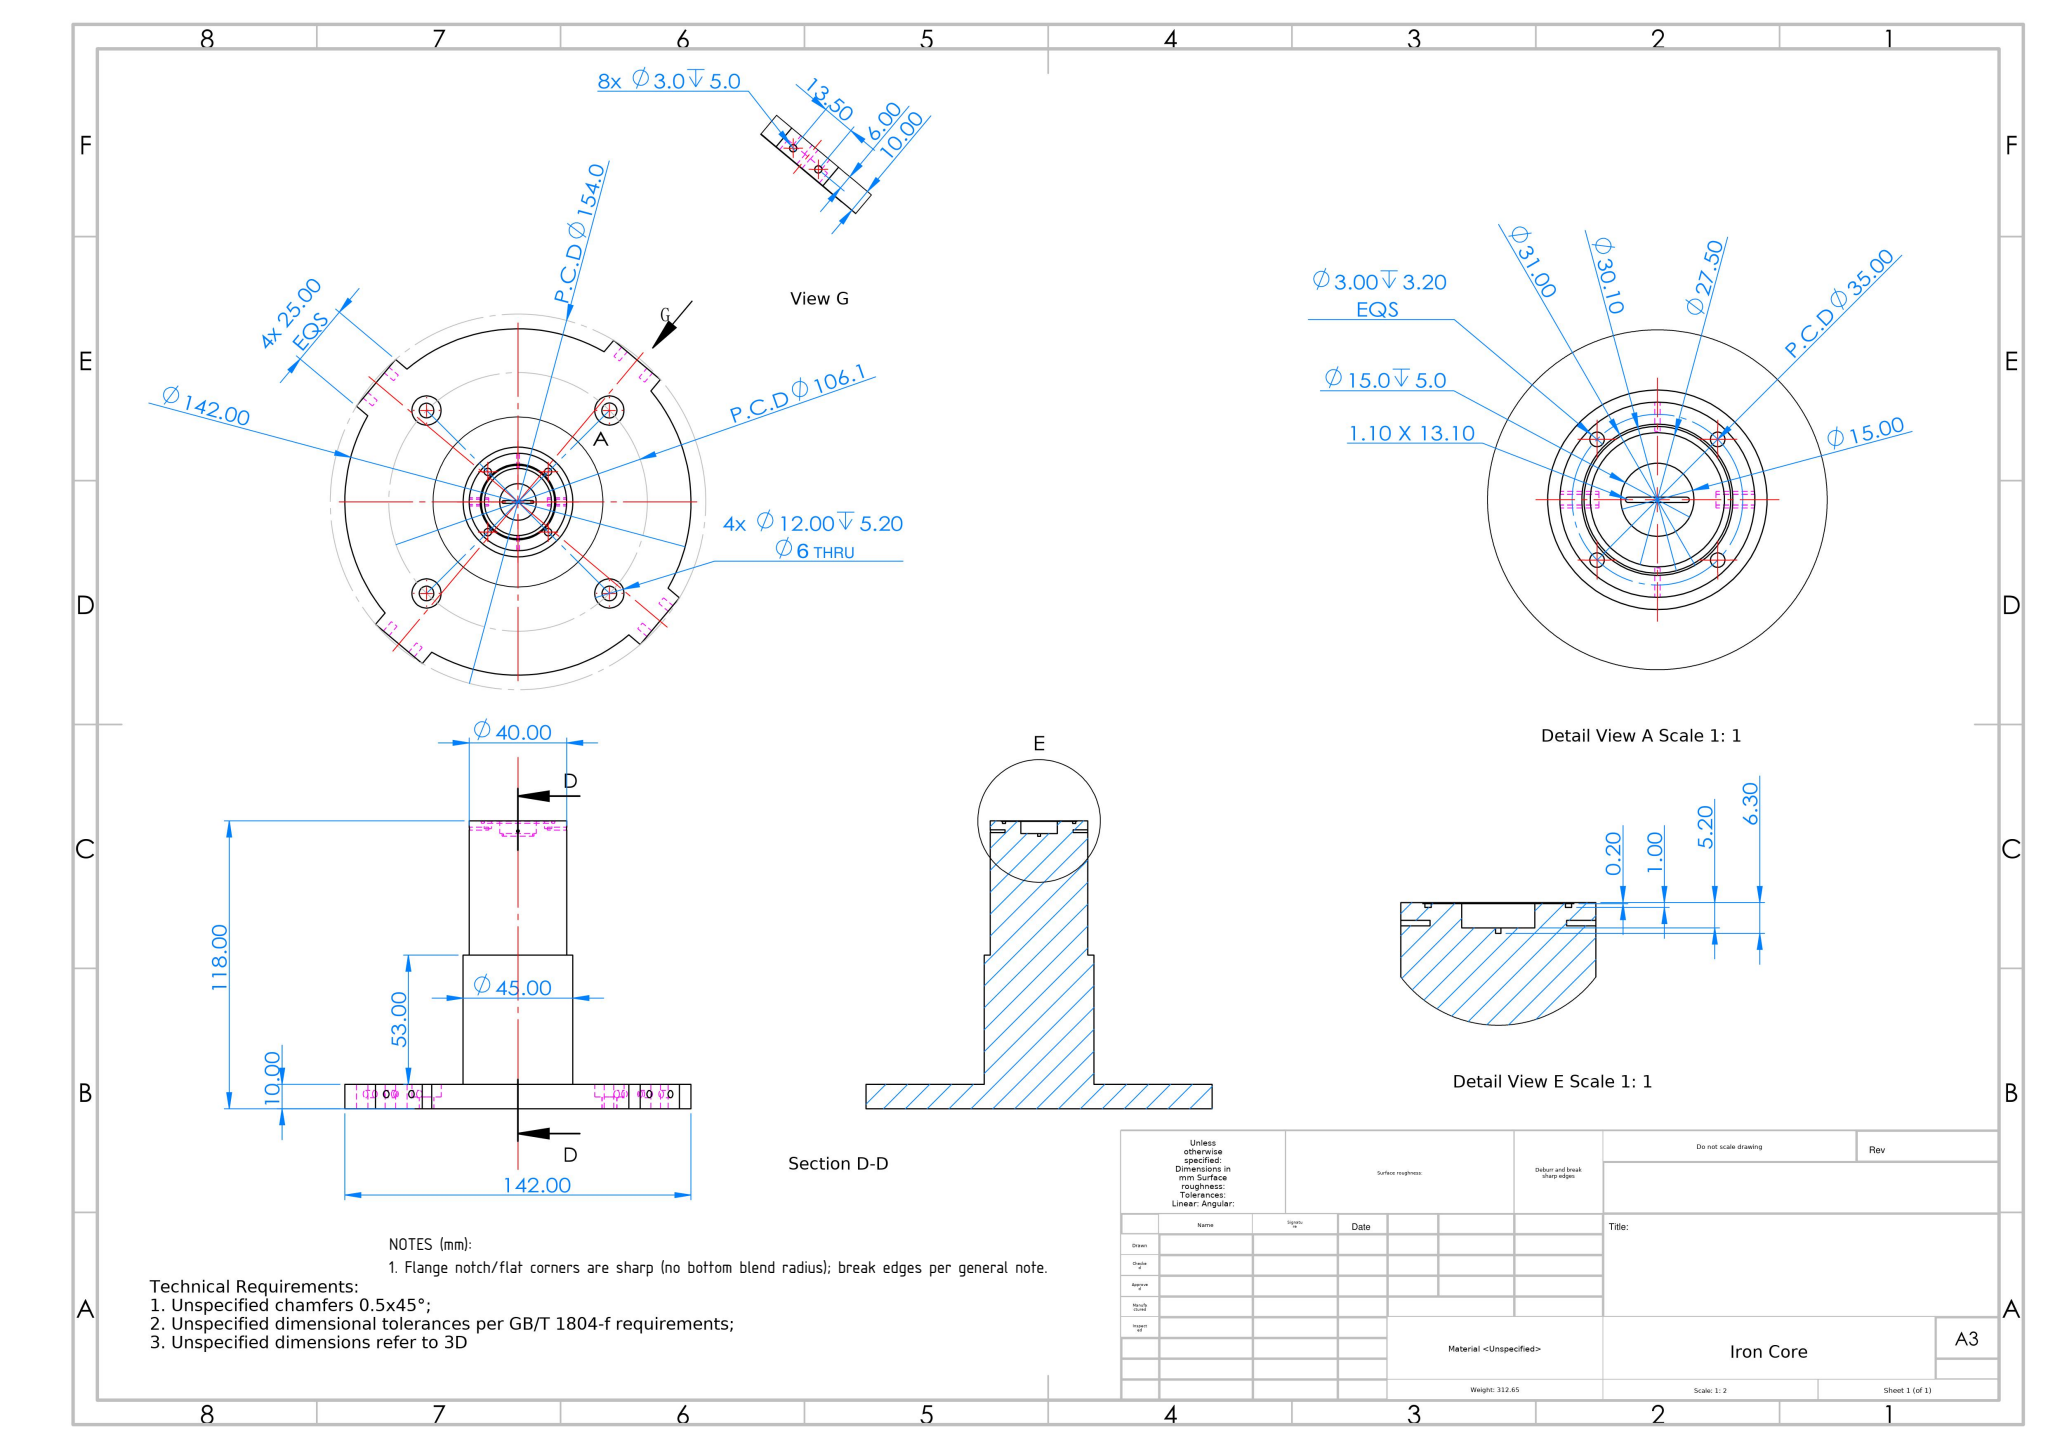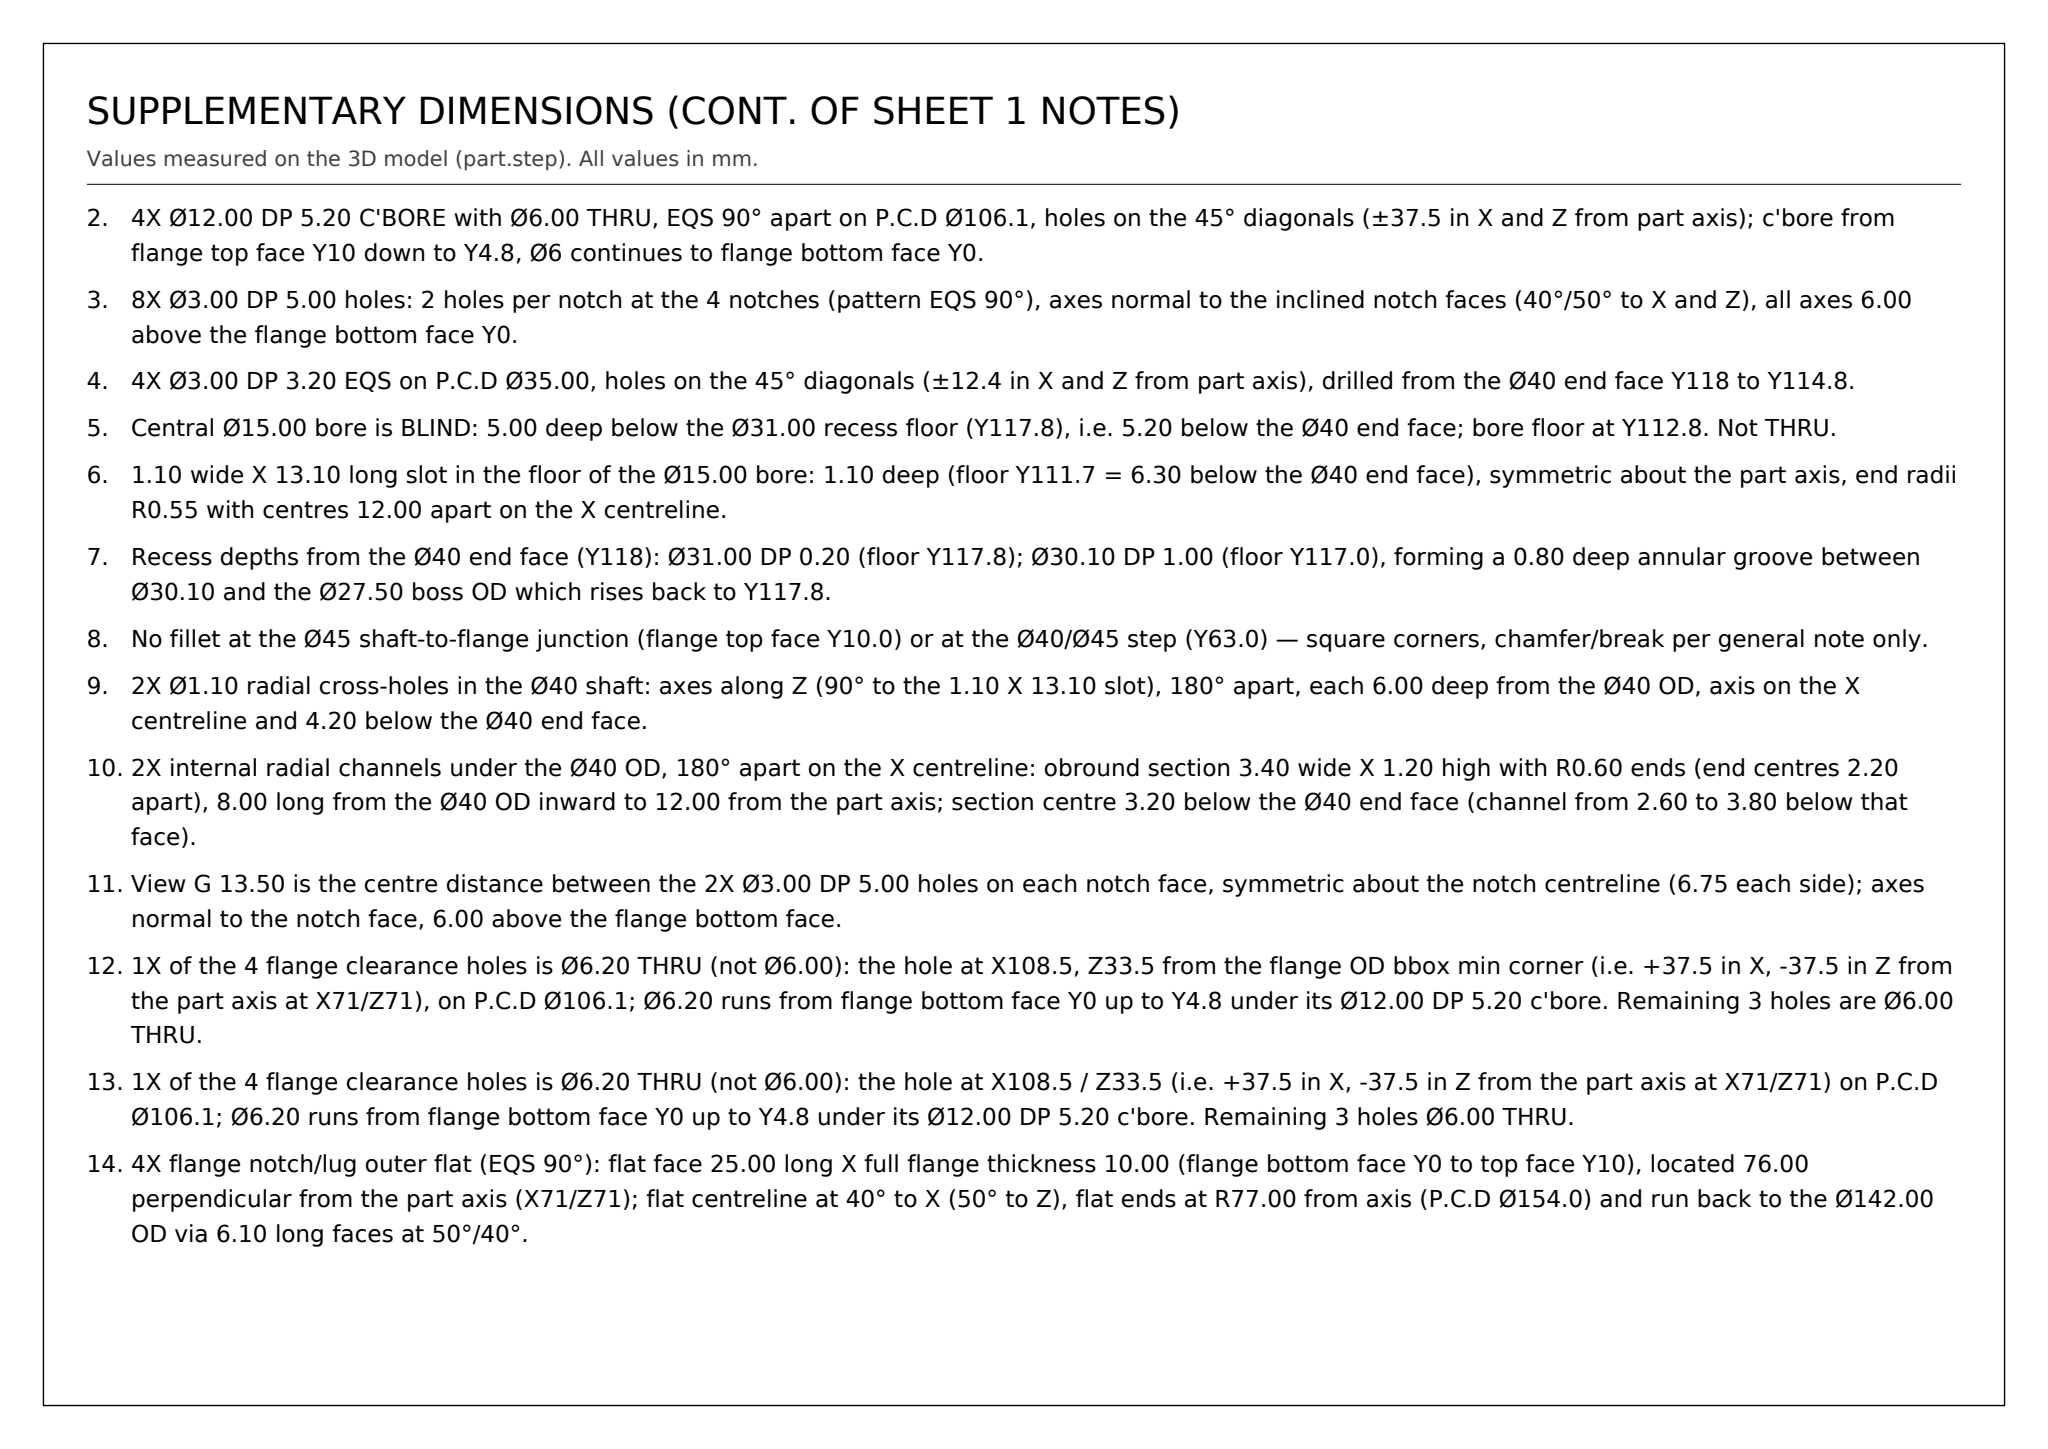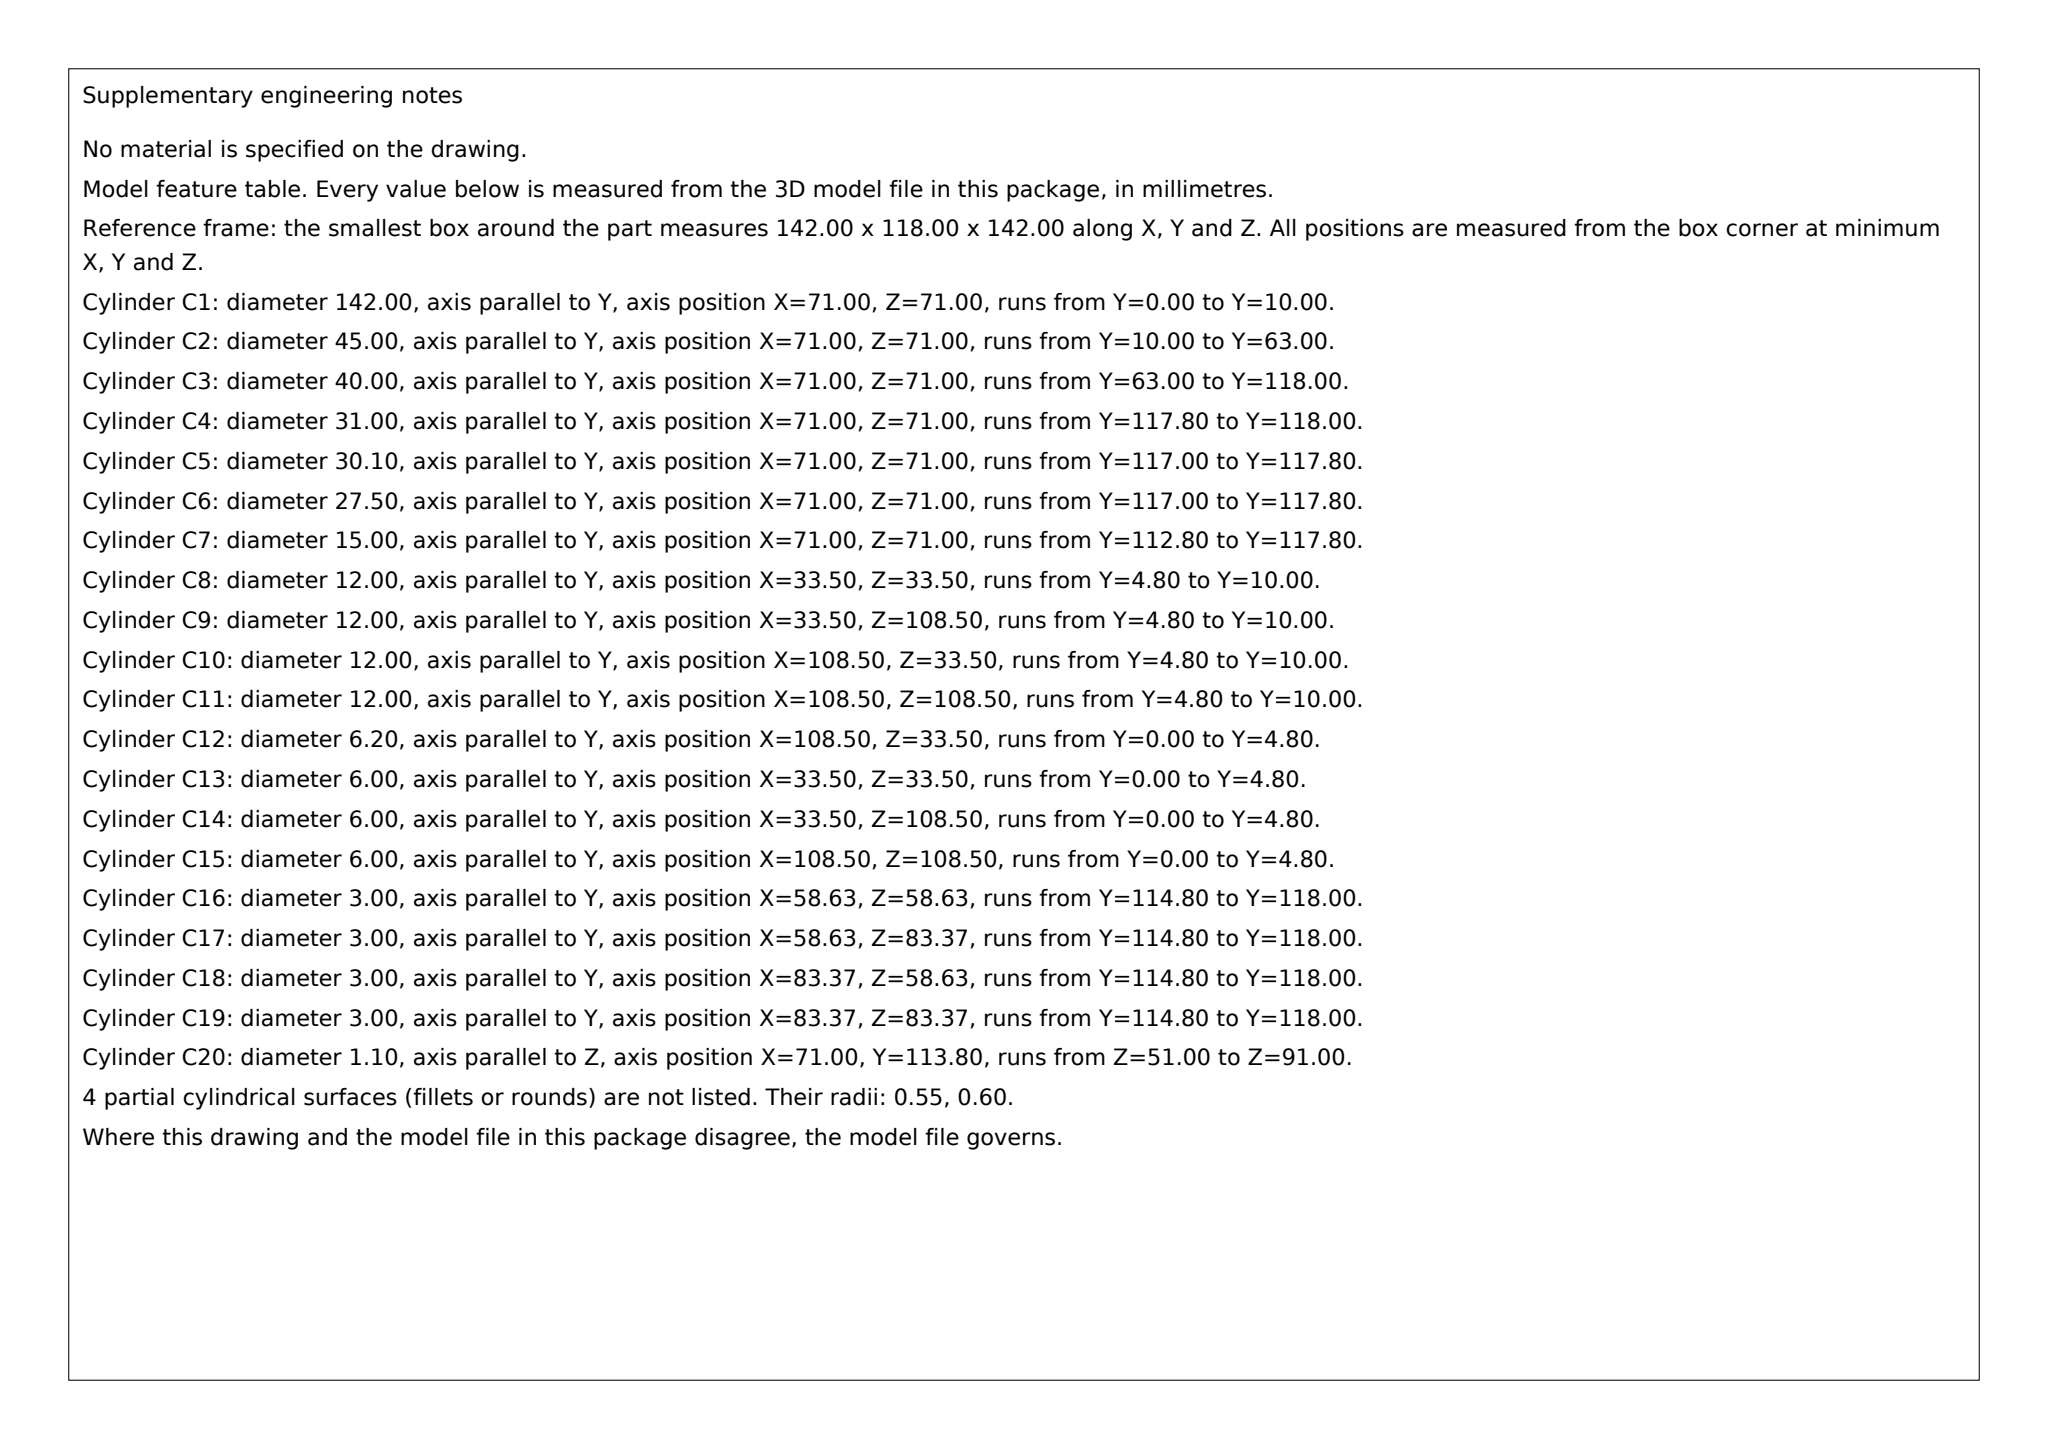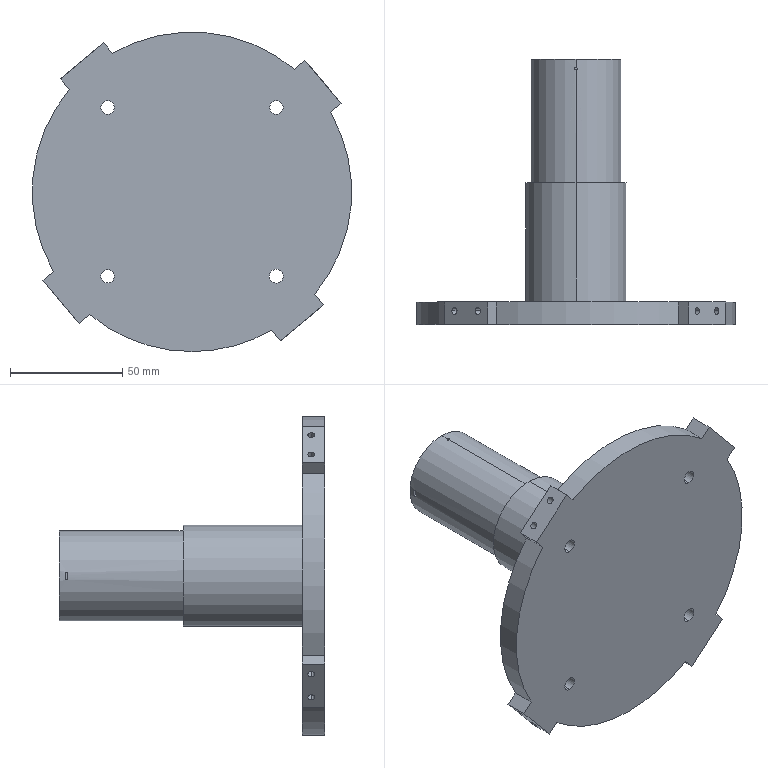Part | SolidWorks | mm | 1 solid | 116 faces | box 142 x 118 x 142 mm | volume 312651 mm3 | cylinder 69 | plane 47 | commonest cylinder face diameters 3 x24 12 x8 1.1 x6 1.2 x6 6 x6 142 x5 15 x2 31 x2
Drawing notes:
Flange notch/flat corners are sharp (no bottom blend radius); break edges per general note. | from the solid: tori[minor_r,major_r] list is empty (no blends anywhere in model)
4X Ø12.00 DP 5.20 C'BORE with Ø6.00 THRU, EQS 90° apart on P.C.D Ø106.1, holes on the 45° diagonals (±37.5 in X and Z from part axis); c'bore from flange top face Y10 down to Y4.8, Ø6 continues to flange bottom face Y0. | from the solid: hole/bore 12.0 axis y at (108.5,108.5),(108.5,33.5),(33.5,108.5),(33.5,33.5) from 4.8 to 10.0; hole/bore 6.0 same centres from 0.0 to 4.8
8X Ø3.00 DP 5.00 holes: 2 holes per notch at the 4 notches (pattern EQS 90°), axes normal to the inclined notch faces (40°/50° to X and Z), all axes 6.00 above the flange bottom face Y0. | from the solid: 8 x hole/bore dia 3.0 'inclined' all with axis_pos y = 6.0, in 4 symmetric pairs (e.g. x=111.5 & 121.8; z=111.5 & 121.8; x=20.2 & 30.5; z=20.2 & 30.5)
4X Ø3.00 DP 3.20 EQS on P.C.D Ø35.00, holes on the 45° diagonals (±12.4 in X and Z from part axis), drilled from the Ø40 end face Y118 to Y114.8. | from the solid: hole/bore 3.0 axis y at (58.6,58.6),(58.6,83.4),(83.4,58.6),(83.4,83.4) from 114.8 to 118.0
Central Ø15.00 bore is BLIND: 5.00 deep below the Ø31.00 recess floor (Y117.8), i.e. 5.20 below the Ø40 end face; bore floor at Y112.8. Not THRU. | from the solid: hole/bore 15.0 axis y at (71,71) from 112.8 to 117.8; Ø40 end face plane y=118.0
1.10 wide X 13.10 long slot in the floor of the Ø15.00 bore: 1.10 deep (floor Y111.7 = 6.30 below the Ø40 end face), symmetric about the part axis, end radii R0.55 with centres 12.00 apart on the X centreline. | from the solid: concave arcs dia 1.1 axis y at (65,71) and (77,71) from 111.7 to 112.8; plane y=111.7 extent x[64.4,77.6], z[70.4,71.6]
Recess depths from the Ø40 end face (Y118): Ø31.00 DP 0.20 (floor Y117.8); Ø30.10 DP 1.00 (floor Y117.0), forming a 0.80 deep annular groove between Ø30.10 and the Ø27.50 boss OD which rises back to Y117.8. | from the solid: hole/bore 31.0 from 117.8 to 118.0; hole/bore 30.1 from 117.0 to 117.8; boss/shaft 27.5 from 117.0 to 117.8; planes y=117.0, y=117.8, y=118.0
No fillet at the Ø45 shaft-to-flange junction (flange top face Y10.0) or at the Ø40/Ø45 step (Y63.0) — square corners, chamfer/break per general note only. | from the solid: planes y=10.0 and y=63.0 meet cylinders dia 45 (10.0-63.0) and dia 40 (63.0-118.0); tori list empty
2X Ø1.10 radial cross-holes in the Ø40 shaft: axes along Z (90° to the 1.10 X 13.10 slot), 180° apart, each 6.00 deep from the Ø40 OD, axis on the X centreline and 4.20 below the Ø40 end face. | from the solid: hole/bore dia 1.1 axis z at [71.0, 113.8] from 51.0 to 57.0 and from 85.0 to 91.0 (Ø40 OD at z51/z91, end face Y118)
2X internal radial channels under the Ø40 OD, 180° apart on the X centreline: obround section 3.40 wide X 1.20 high with R0.60 ends (end centres 2.20 apart), 8.00 long from the Ø40 OD inward to 12.00 from the part axis; section centre 3.20 below the Ø40 end face (channel from 2.60 to 3.80 below that face). | from the solid: planes y114.2 and y115.4 extent x[51,59] and x[83,91], z[69.9,72.1]; end planes x59 and x83 extent z[69.3,72.7]; arcs dia 1.2 axis x at y114.8, z69.9 and z72.1, from x51 to x59 / x83 to x91
View G 13.50 is the centre distance between the 2X Ø3.00 DP 5.00 holes on each notch face, symmetric about the notch centreline (6.75 each side); axes normal to the notch face, 6.00 above the flange bottom face. | from the solid: inclined Ø3.0 hole axis pairs e.g. [111.5,6.0] and [121.8,6.0] with runs 7.5-13.2 and 16.2-21.9 => 13.48 centre spacing, all at y=6.0
1X of the 4 flange clearance holes is Ø6.20 THRU (not Ø6.00): the hole at X108.5, Z33.5 from the flange OD bbox min corner (i.e. +37.5 in X, -37.5 in Z from the part axis at X71/Z71), on P.C.D Ø106.1; Ø6.20 runs from flange bottom face Y0 up to Y4.8 under its Ø12.00 DP 5.20 c'bore. Remaining 3 holes are Ø6.00 THRU. | from the solid: cylinders: ["hole/bore", 6.2, "y", [108.5, null, 33.5], from 0.0 to 4.8, 360] vs three ["hole/bore", 6.0, "y", ...] at [108.5,108.5], [33.5,108.5], [33.5,33.5]; c'bore ["hole/bore",12.0,"y",[108.5,null,33.5],from 4.8 to 10.0]
1X of the 4 flange clearance holes is Ø6.20 THRU (not Ø6.00): the hole at X108.5 / Z33.5 (i.e. +37.5 in X, -37.5 in Z from the part axis at X71/Z71) on P.C.D Ø106.1; Ø6.20 runs from flange bottom face Y0 up to Y4.8 under its Ø12.00 DP 5.20 c'bore. Remaining 3 holes Ø6.00 THRU. | from the solid: cylinders: ['hole/bore', 6.2, 'y', [108.5, null, 33.5], 'from', 0.0, 'to', 4.8, 360] vs three ['hole/bore', 6.0, 'y', [108.5,108.5]/[33.5,108.5]/[33.5,33.5], 0.0 to 4.8]; ['hole/bore', 12.0, 'y', [108.5, null, 33.5], 4.8 to 10.0]
4X flange notch/lug outer flat (EQS 90°): flat face 25.00 long X full flange thickness 10.00 (flange bottom face Y0 to top face Y10), located 76.00 perpendicular from the part axis (X71/Z71); flat centreline at 40° to X (50° to Z), flat ends at R77.00 from axis (P.C.D Ø154.0) and run back to the Ø142.00 OD via 6.10 long faces at 50°/40°. | from the solid: inclined_planes: 4X face size 16.1x10.0x19.2 (in-plane length 25.06) at angle_to_xyz_axes [40,90,50]/[50,90,40], e.g. bbox_from [4.7,0.0,12.6] — face midpoint 76.0 from axis X71/Z71, corners at 77.0; adjacent 4.7x10.0x3.9 faces (length 6.1) end on the convex arc dia 142 (arc_deg 279) at r=71.0